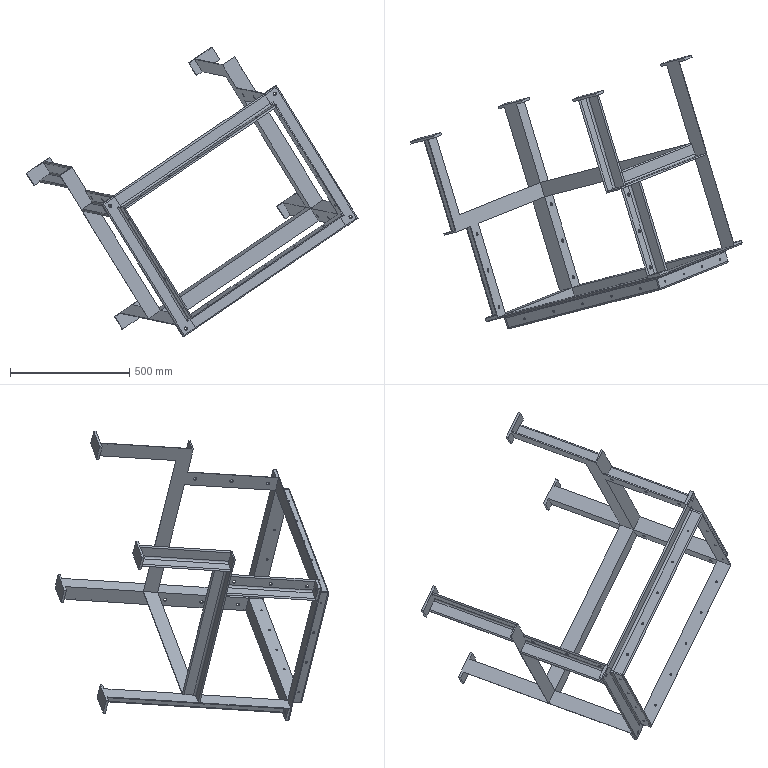Component | SolidWorks | CrusherFrame-1 | 3 solids | 223 faces | volume 6302922 mm3 | cylinder 119 | plane 104 | commonest cylinder face diameters 8 x36 12 x34 14 x32 18 x17